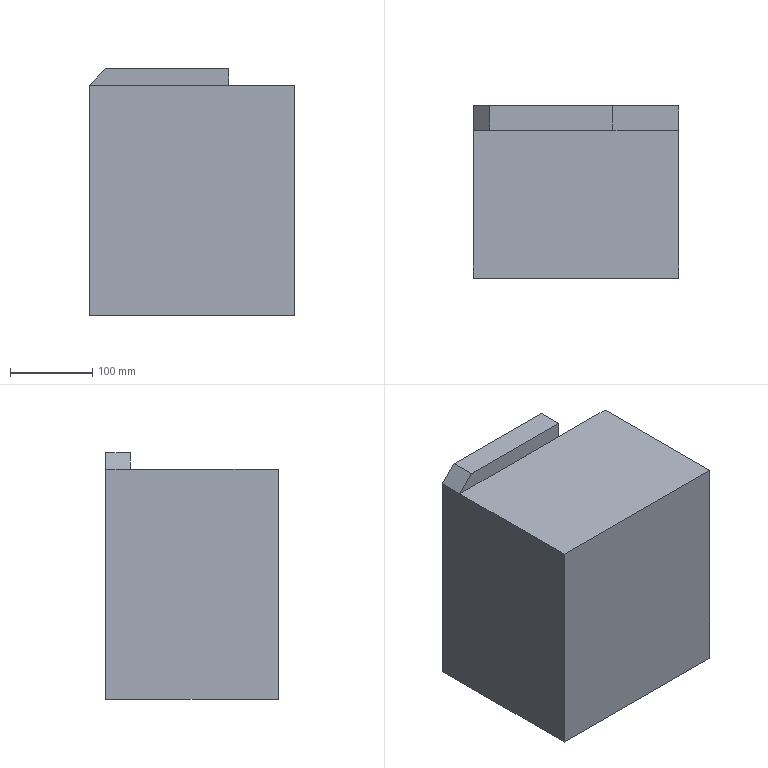Component | SolidWorks | -3[1]-1 | 1 solid | 15 faces | box 250 x 210 x 300 mm | volume 14226823 mm3 | plane 13 | cylinder 2 | commonest cylinder face diameters 27 x2
STEP:
#1=COLOUR_RGB('',0.7922,0.8196,0.9333);
#2=FILL_AREA_STYLE_COLOUR('',#1);
#3=FILL_AREA_STYLE('',(#2));
#4=SURFACE_STYLE_FILL_AREA(#3);
#5=SURFACE_SIDE_STYLE('',(#4));
#6=SURFACE_STYLE_USAGE(.BOTH.,#5);
#7=PRESENTATION_STYLE_ASSIGNMENT((#6));
#8=CARTESIAN_POINT('',(-19.685,-89.764,-4.39));
#9=VERTEX_POINT('',#8);
#10=CARTESIAN_POINT('',(-19.685,-89.764,-5.453));
#11=VERTEX_POINT('',#10);
#12=CARTESIAN_POINT('',(-19.685,-89.764,-4.921));
#13=DIRECTION('',(0.,-1.,0.));
#14=DIRECTION('',(0.,0.,-1.));
#15=AXIS2_PLACEMENT_3D('',#12,#13,#14);
#16=CIRCLE('',#15,0.5315);
#17=EDGE_CURVE('',#9,#11,#16,.T.);
#18=ORIENTED_EDGE('',*,*,#17,.T.);
#19=CARTESIAN_POINT('',(-19.685,-88.583,-5.453));
#20=VERTEX_POINT('',#19);
#21=CARTESIAN_POINT('',(-19.685,-89.764,-5.453));
#22=DIRECTION('',(0.,1.,0.));
#23=VECTOR('',#22,39.37);
#24=LINE('',#21,#23);
#25=EDGE_CURVE('',#11,#20,#24,.T.);
#26=ORIENTED_EDGE('',*,*,#25,.T.);
#27=CARTESIAN_POINT('',(-19.685,-88.583,-4.39));
#28=VERTEX_POINT('',#27);
#29=CARTESIAN_POINT('',(-19.685,-88.583,-4.921));
#30=DIRECTION('',(0.,-1.,0.));
#31=DIRECTION('',(0.,0.,-1.));
#32=AXIS2_PLACEMENT_3D('',#29,#30,#31);
#33=CIRCLE('',#32,0.5315);
#34=EDGE_CURVE('',#28,#20,#33,.T.);
#35=ORIENTED_EDGE('',*,*,#34,.F.);
#36=CARTESIAN_POINT('',(-19.685,-89.764,-4.39));
#37=DIRECTION('',(0.,1.,0.));
#38=VECTOR('',#37,39.37);
#39=LINE('',#36,#38);
#40=EDGE_CURVE('',#9,#28,#39,.T.);
#41=ORIENTED_EDGE('',*,*,#40,.F.);
#42=EDGE_LOOP('',(#18,#26,#35,#41));
#43=FACE_OUTER_BOUND('',#42,.T.);
#44=CARTESIAN_POINT('',(-19.685,-89.764,-4.921));
#45=DIRECTION('',(0.,1.,0.));
#46=DIRECTION('',(0.,0.,-1.));
#47=AXIS2_PLACEMENT_3D('',#44,#45,#46);
#48=CYLINDRICAL_SURFACE('',#47,0.5315);
#49=ADVANCED_FACE('',(#43),#48,.F.);
#50=CARTESIAN_POINT('',(-14.961,-89.764,2.165));
#51=VERTEX_POINT('',#50);
#52=CARTESIAN_POINT('',(-21.654,-89.764,2.165));
#53=VERTEX_POINT('',#52);
#54=CARTESIAN_POINT('',(-21.654,-89.764,2.165));
#55=DIRECTION('',(-1.,0.,0.));
#56=VECTOR('',#55,39.37);
#57=LINE('',#54,#56);
#58=EDGE_CURVE('',#51,#53,#57,.T.);
#59=ORIENTED_EDGE('',*,*,#58,.F.);
#60=CARTESIAN_POINT('',(-14.961,-89.764,2.953));
#61=VERTEX_POINT('',#60);
#62=CARTESIAN_POINT('',(-14.961,-89.764,2.953));
#63=DIRECTION('',(-0.,0.,1.));
#64=VECTOR('',#63,39.37);
#65=LINE('',#62,#64);
#66=EDGE_CURVE('',#51,#61,#65,.T.);
#67=ORIENTED_EDGE('',*,*,#66,.T.);
#68=CARTESIAN_POINT('',(-20.866,-89.764,2.953));
#69=VERTEX_POINT('',#68);
#70=CARTESIAN_POINT('',(-20.866,-89.764,2.953));
#71=DIRECTION('',(-1.,0.,0.));
#72=VECTOR('',#71,39.37);
#73=LINE('',#70,#72);
#74=EDGE_CURVE('',#61,#69,#73,.T.);
#75=ORIENTED_EDGE('',*,*,#74,.T.);
#76=CARTESIAN_POINT('',(-21.654,-89.764,2.165));
#77=DIRECTION('',(-0.7071,0.,-0.7071));
#78=VECTOR('',#77,39.37);
#79=LINE('',#76,#78);
#80=EDGE_CURVE('',#69,#53,#79,.T.);
#81=ORIENTED_EDGE('',*,*,#80,.T.);
#82=EDGE_LOOP('',(#59,#67,#75,#81));
#83=FACE_OUTER_BOUND('',#82,.T.);
#84=CARTESIAN_POINT('',(-21.654,-89.764,-8.858));
#85=DIRECTION('',(0.,1.,0.));
#86=DIRECTION('',(0.,0.,-1.));
#87=AXIS2_PLACEMENT_3D('',#84,#85,#86);
#88=PLANE('',#87);
#89=ADVANCED_FACE('',(#83),#88,.F.);
#90=CARTESIAN_POINT('',(-21.654,-88.583,-8.858));
#91=VERTEX_POINT('',#90);
#92=CARTESIAN_POINT('',(-11.811,-88.583,-8.858));
#93=VERTEX_POINT('',#92);
#94=CARTESIAN_POINT('',(-11.811,-88.583,-8.858));
#95=DIRECTION('',(1.,0.,0.));
#96=VECTOR('',#95,39.37);
#97=LINE('',#94,#96);
#98=EDGE_CURVE('',#91,#93,#97,.T.);
#99=ORIENTED_EDGE('',*,*,#98,.F.);
#100=CARTESIAN_POINT('',(-21.654,-88.583,2.165));
#101=VERTEX_POINT('',#100);
#102=CARTESIAN_POINT('',(-21.654,-88.583,-8.858));
#103=DIRECTION('',(0.,0.,-1.));
#104=VECTOR('',#103,39.37);
#105=LINE('',#102,#104);
#106=EDGE_CURVE('',#101,#91,#105,.T.);
#107=ORIENTED_EDGE('',*,*,#106,.F.);
#108=CARTESIAN_POINT('',(-20.866,-88.583,2.953));
#109=VERTEX_POINT('',#108);
#110=CARTESIAN_POINT('',(-21.654,-88.583,2.165));
#111=DIRECTION('',(-0.7071,0.,-0.7071));
#112=VECTOR('',#111,39.37);
#113=LINE('',#110,#112);
#114=EDGE_CURVE('',#109,#101,#113,.T.);
#115=ORIENTED_EDGE('',*,*,#114,.F.);
#116=CARTESIAN_POINT('',(-14.961,-88.583,2.953));
#117=VERTEX_POINT('',#116);
#118=CARTESIAN_POINT('',(-20.866,-88.583,2.953));
#119=DIRECTION('',(-1.,0.,0.));
#120=VECTOR('',#119,39.37);
#121=LINE('',#118,#120);
#122=EDGE_CURVE('',#117,#109,#121,.T.);
#123=ORIENTED_EDGE('',*,*,#122,.F.);
#124=CARTESIAN_POINT('',(-14.961,-88.583,-6.89));
#125=VERTEX_POINT('',#124);
#126=CARTESIAN_POINT('',(-14.961,-88.583,2.953));
#127=DIRECTION('',(-0.,0.,1.));
#128=VECTOR('',#127,39.37);
#129=LINE('',#126,#128);
#130=EDGE_CURVE('',#125,#117,#129,.T.);
#131=ORIENTED_EDGE('',*,*,#130,.F.);
#132=CARTESIAN_POINT('',(-11.811,-88.583,-6.89));
#133=VERTEX_POINT('',#132);
#134=CARTESIAN_POINT('',(-14.961,-88.583,-6.89));
#135=DIRECTION('',(-1.,0.,0.));
#136=VECTOR('',#135,39.37);
#137=LINE('',#134,#136);
#138=EDGE_CURVE('',#133,#125,#137,.T.);
#139=ORIENTED_EDGE('',*,*,#138,.F.);
#140=CARTESIAN_POINT('',(-11.811,-88.583,-6.89));
#141=DIRECTION('',(0.,0.,1.));
#142=VECTOR('',#141,39.37);
#143=LINE('',#140,#142);
#144=EDGE_CURVE('',#93,#133,#143,.T.);
#145=ORIENTED_EDGE('',*,*,#144,.F.);
#146=EDGE_LOOP('',(#99,#107,#115,#123,#131,#139,#145));
#147=FACE_OUTER_BOUND('',#146,.T.);
#148=ORIENTED_EDGE('',*,*,#34,.T.);
#149=CARTESIAN_POINT('',(-19.685,-88.583,-4.921));
#150=DIRECTION('',(0.,-1.,0.));
#151=DIRECTION('',(0.,0.,-1.));
#152=AXIS2_PLACEMENT_3D('',#149,#150,#151);
#153=CIRCLE('',#152,0.5315);
#154=EDGE_CURVE('',#20,#28,#153,.T.);
#155=ORIENTED_EDGE('',*,*,#154,.T.);
#156=EDGE_LOOP('',(#148,#155));
#157=FACE_BOUND('',#156,.T.);
#158=CARTESIAN_POINT('',(-21.654,-88.583,-8.858));
#159=DIRECTION('',(0.,1.,0.));
#160=DIRECTION('',(0.,0.,-1.));
#161=AXIS2_PLACEMENT_3D('',#158,#159,#160);
#162=PLANE('',#161);
#163=ADVANCED_FACE('',(#147,#157),#162,.T.);
#164=ORIENTED_EDGE('',*,*,#98,.T.);
#165=CARTESIAN_POINT('',(-11.811,-96.85,-8.858));
#166=VERTEX_POINT('',#165);
#167=CARTESIAN_POINT('',(-11.811,-89.764,-8.858));
#168=DIRECTION('',(0.,1.,0.));
#169=VECTOR('',#168,39.37);
#170=LINE('',#167,#169);
#171=EDGE_CURVE('',#166,#93,#170,.T.);
#172=ORIENTED_EDGE('',*,*,#171,.F.);
#173=CARTESIAN_POINT('',(-21.654,-96.85,-8.858));
#174=VERTEX_POINT('',#173);
#175=CARTESIAN_POINT('',(-21.654,-96.85,-8.858));
#176=DIRECTION('',(1.,0.,0.));
#177=VECTOR('',#176,39.37);
#178=LINE('',#175,#177);
#179=EDGE_CURVE('',#174,#166,#178,.T.);
#180=ORIENTED_EDGE('',*,*,#179,.F.);
#181=CARTESIAN_POINT('',(-21.654,-89.764,-8.858));
#182=DIRECTION('',(0.,1.,0.));
#183=VECTOR('',#182,39.37);
#184=LINE('',#181,#183);
#185=EDGE_CURVE('',#174,#91,#184,.T.);
#186=ORIENTED_EDGE('',*,*,#185,.T.);
#187=EDGE_LOOP('',(#164,#172,#180,#186));
#188=FACE_OUTER_BOUND('',#187,.T.);
#189=CARTESIAN_POINT('',(-11.811,-89.764,-8.858));
#190=DIRECTION('',(0.,0.,1.));
#191=DIRECTION('',(-1.,0.,0.));
#192=AXIS2_PLACEMENT_3D('',#189,#190,#191);
#193=PLANE('',#192);
#194=ADVANCED_FACE('',(#188),#193,.F.);
#195=ORIENTED_EDGE('',*,*,#144,.T.);
#196=CARTESIAN_POINT('',(-11.811,-89.764,-6.89));
#197=VERTEX_POINT('',#196);
#198=CARTESIAN_POINT('',(-11.811,-89.764,-6.89));
#199=DIRECTION('',(0.,1.,0.));
#200=VECTOR('',#199,39.37);
#201=LINE('',#198,#200);
#202=EDGE_CURVE('',#197,#133,#201,.T.);
#203=ORIENTED_EDGE('',*,*,#202,.F.);
#204=CARTESIAN_POINT('',(-11.811,-89.764,2.165));
#205=VERTEX_POINT('',#204);
#206=CARTESIAN_POINT('',(-11.811,-89.764,2.165));
#207=DIRECTION('',(0.,0.,1.));
#208=VECTOR('',#207,39.37);
#209=LINE('',#206,#208);
#210=EDGE_CURVE('',#197,#205,#209,.T.);
#211=ORIENTED_EDGE('',*,*,#210,.T.);
#212=CARTESIAN_POINT('',(-11.811,-96.85,2.165));
#213=VERTEX_POINT('',#212);
#214=CARTESIAN_POINT('',(-11.811,-96.85,2.165));
#215=DIRECTION('',(0.,1.,0.));
#216=VECTOR('',#215,39.37);
#217=LINE('',#214,#216);
#218=EDGE_CURVE('',#213,#205,#217,.T.);
#219=ORIENTED_EDGE('',*,*,#218,.F.);
#220=CARTESIAN_POINT('',(-11.811,-96.85,2.165));
#221=DIRECTION('',(0.,0.,1.));
#222=VECTOR('',#221,39.37);
#223=LINE('',#220,#222);
#224=EDGE_CURVE('',#166,#213,#223,.T.);
#225=ORIENTED_EDGE('',*,*,#224,.F.);
#226=ORIENTED_EDGE('',*,*,#171,.T.);
#227=EDGE_LOOP('',(#195,#203,#211,#219,#225,#226));
#228=FACE_OUTER_BOUND('',#227,.T.);
#229=CARTESIAN_POINT('',(-11.811,-89.764,-6.89));
#230=DIRECTION('',(-1.,0.,0.));
#231=DIRECTION('',(0.,0.,-1.));
#232=AXIS2_PLACEMENT_3D('',#229,#230,#231);
#233=PLANE('',#232);
#234=ADVANCED_FACE('',(#228),#233,.F.);
#235=ORIENTED_EDGE('',*,*,#138,.T.);
#236=CARTESIAN_POINT('',(-14.961,-89.764,-6.89));
#237=VERTEX_POINT('',#236);
#238=CARTESIAN_POINT('',(-14.961,-89.764,-6.89));
#239=DIRECTION('',(0.,1.,0.));
#240=VECTOR('',#239,39.37);
#241=LINE('',#238,#240);
#242=EDGE_CURVE('',#237,#125,#241,.T.);
#243=ORIENTED_EDGE('',*,*,#242,.F.);
#244=CARTESIAN_POINT('',(-14.961,-89.764,-6.89));
#245=DIRECTION('',(-1.,0.,0.));
#246=VECTOR('',#245,39.37);
#247=LINE('',#244,#246);
#248=EDGE_CURVE('',#197,#237,#247,.T.);
#249=ORIENTED_EDGE('',*,*,#248,.F.);
#250=ORIENTED_EDGE('',*,*,#202,.T.);
#251=EDGE_LOOP('',(#235,#243,#249,#250));
#252=FACE_OUTER_BOUND('',#251,.T.);
#253=CARTESIAN_POINT('',(-14.961,-89.764,-6.89));
#254=DIRECTION('',(0.,0.,-1.));
#255=DIRECTION('',(1.,0.,0.));
#256=AXIS2_PLACEMENT_3D('',#253,#254,#255);
#257=PLANE('',#256);
#258=ADVANCED_FACE('',(#252),#257,.F.);
#259=ORIENTED_EDGE('',*,*,#130,.T.);
#260=CARTESIAN_POINT('',(-14.961,-89.764,2.953));
#261=DIRECTION('',(0.,1.,0.));
#262=VECTOR('',#261,39.37);
#263=LINE('',#260,#262);
#264=EDGE_CURVE('',#61,#117,#263,.T.);
#265=ORIENTED_EDGE('',*,*,#264,.F.);
#266=ORIENTED_EDGE('',*,*,#66,.F.);
#267=CARTESIAN_POINT('',(-14.961,-89.764,2.953));
#268=DIRECTION('',(-0.,0.,1.));
#269=VECTOR('',#268,39.37);
#270=LINE('',#267,#269);
#271=EDGE_CURVE('',#237,#51,#270,.T.);
#272=ORIENTED_EDGE('',*,*,#271,.F.);
#273=ORIENTED_EDGE('',*,*,#242,.T.);
#274=EDGE_LOOP('',(#259,#265,#266,#272,#273));
#275=FACE_OUTER_BOUND('',#274,.T.);
#276=CARTESIAN_POINT('',(-14.961,-89.764,2.953));
#277=DIRECTION('',(-1.,0.,-0.));
#278=DIRECTION('',(0.,0.,-1.));
#279=AXIS2_PLACEMENT_3D('',#276,#277,#278);
#280=PLANE('',#279);
#281=ADVANCED_FACE('',(#275),#280,.F.);
#282=ORIENTED_EDGE('',*,*,#122,.T.);
#283=CARTESIAN_POINT('',(-20.866,-89.764,2.953));
#284=DIRECTION('',(0.,1.,0.));
#285=VECTOR('',#284,39.37);
#286=LINE('',#283,#285);
#287=EDGE_CURVE('',#69,#109,#286,.T.);
#288=ORIENTED_EDGE('',*,*,#287,.F.);
#289=ORIENTED_EDGE('',*,*,#74,.F.);
#290=ORIENTED_EDGE('',*,*,#264,.T.);
#291=EDGE_LOOP('',(#282,#288,#289,#290));
#292=FACE_OUTER_BOUND('',#291,.T.);
#293=CARTESIAN_POINT('',(-20.866,-89.764,2.953));
#294=DIRECTION('',(0.,0.,-1.));
#295=DIRECTION('',(1.,0.,0.));
#296=AXIS2_PLACEMENT_3D('',#293,#294,#295);
#297=PLANE('',#296);
#298=ADVANCED_FACE('',(#292),#297,.F.);
#299=ORIENTED_EDGE('',*,*,#114,.T.);
#300=CARTESIAN_POINT('',(-21.654,-89.764,2.165));
#301=DIRECTION('',(0.,1.,0.));
#302=VECTOR('',#301,39.37);
#303=LINE('',#300,#302);
#304=EDGE_CURVE('',#53,#101,#303,.T.);
#305=ORIENTED_EDGE('',*,*,#304,.F.);
#306=ORIENTED_EDGE('',*,*,#80,.F.);
#307=ORIENTED_EDGE('',*,*,#287,.T.);
#308=EDGE_LOOP('',(#299,#305,#306,#307));
#309=FACE_OUTER_BOUND('',#308,.T.);
#310=CARTESIAN_POINT('',(-21.654,-89.764,2.165));
#311=DIRECTION('',(0.7071,0.,-0.7071));
#312=DIRECTION('',(0.7071,0.,0.7071));
#313=AXIS2_PLACEMENT_3D('',#310,#311,#312);
#314=PLANE('',#313);
#315=ADVANCED_FACE('',(#309),#314,.F.);
#316=ORIENTED_EDGE('',*,*,#106,.T.);
#317=ORIENTED_EDGE('',*,*,#185,.F.);
#318=CARTESIAN_POINT('',(-21.654,-96.85,2.165));
#319=VERTEX_POINT('',#318);
#320=CARTESIAN_POINT('',(-21.654,-96.85,2.165));
#321=DIRECTION('',(0.,0.,-1.));
#322=VECTOR('',#321,39.37);
#323=LINE('',#320,#322);
#324=EDGE_CURVE('',#319,#174,#323,.T.);
#325=ORIENTED_EDGE('',*,*,#324,.F.);
#326=CARTESIAN_POINT('',(-21.654,-96.85,2.165));
#327=DIRECTION('',(0.,1.,0.));
#328=VECTOR('',#327,39.37);
#329=LINE('',#326,#328);
#330=EDGE_CURVE('',#319,#53,#329,.T.);
#331=ORIENTED_EDGE('',*,*,#330,.T.);
#332=ORIENTED_EDGE('',*,*,#304,.T.);
#333=EDGE_LOOP('',(#316,#317,#325,#331,#332));
#334=FACE_OUTER_BOUND('',#333,.T.);
#335=CARTESIAN_POINT('',(-21.654,-89.764,-8.858));
#336=DIRECTION('',(1.,0.,0.));
#337=DIRECTION('',(0.,0.,1.));
#338=AXIS2_PLACEMENT_3D('',#335,#336,#337);
#339=PLANE('',#338);
#340=ADVANCED_FACE('',(#334),#339,.F.);
#341=ORIENTED_EDGE('',*,*,#25,.F.);
#342=CARTESIAN_POINT('',(-19.685,-89.764,-4.921));
#343=DIRECTION('',(0.,-1.,0.));
#344=DIRECTION('',(0.,0.,-1.));
#345=AXIS2_PLACEMENT_3D('',#342,#343,#344);
#346=CIRCLE('',#345,0.5315);
#347=EDGE_CURVE('',#11,#9,#346,.T.);
#348=ORIENTED_EDGE('',*,*,#347,.T.);
#349=ORIENTED_EDGE('',*,*,#40,.T.);
#350=ORIENTED_EDGE('',*,*,#154,.F.);
#351=EDGE_LOOP('',(#341,#348,#349,#350));
#352=FACE_OUTER_BOUND('',#351,.T.);
#353=CARTESIAN_POINT('',(-19.685,-89.764,-4.921));
#354=DIRECTION('',(0.,1.,0.));
#355=DIRECTION('',(0.,0.,-1.));
#356=AXIS2_PLACEMENT_3D('',#353,#354,#355);
#357=CYLINDRICAL_SURFACE('',#356,0.5315);
#358=ADVANCED_FACE('',(#352),#357,.F.);
#359=ORIENTED_EDGE('',*,*,#324,.T.);
#360=ORIENTED_EDGE('',*,*,#179,.T.);
#361=ORIENTED_EDGE('',*,*,#224,.T.);
#362=CARTESIAN_POINT('',(-21.654,-96.85,2.165));
#363=DIRECTION('',(-1.,0.,0.));
#364=VECTOR('',#363,39.37);
#365=LINE('',#362,#364);
#366=EDGE_CURVE('',#213,#319,#365,.T.);
#367=ORIENTED_EDGE('',*,*,#366,.T.);
#368=EDGE_LOOP('',(#359,#360,#361,#367));
#369=FACE_OUTER_BOUND('',#368,.T.);
#370=CARTESIAN_POINT('',(0.,-96.85,0.));
#371=DIRECTION('',(0.,-1.,0.));
#372=DIRECTION('',(0.,0.,1.));
#373=AXIS2_PLACEMENT_3D('',#370,#371,#372);
#374=PLANE('',#373);
#375=ADVANCED_FACE('',(#369),#374,.T.);
#376=CARTESIAN_POINT('',(-21.654,-89.764,2.165));
#377=DIRECTION('',(-1.,0.,0.));
#378=VECTOR('',#377,39.37);
#379=LINE('',#376,#378);
#380=EDGE_CURVE('',#205,#51,#379,.T.);
#381=ORIENTED_EDGE('',*,*,#380,.T.);
#382=ORIENTED_EDGE('',*,*,#58,.T.);
#383=ORIENTED_EDGE('',*,*,#330,.F.);
#384=ORIENTED_EDGE('',*,*,#366,.F.);
#385=ORIENTED_EDGE('',*,*,#218,.T.);
#386=EDGE_LOOP('',(#381,#382,#383,#384,#385));
#387=FACE_OUTER_BOUND('',#386,.T.);
#388=CARTESIAN_POINT('',(-21.654,-96.85,2.165));
#389=DIRECTION('',(0.,0.,-1.));
#390=DIRECTION('',(1.,0.,0.));
#391=AXIS2_PLACEMENT_3D('',#388,#389,#390);
#392=PLANE('',#391);
#393=ADVANCED_FACE('',(#387),#392,.F.);
#394=ORIENTED_EDGE('',*,*,#210,.F.);
#395=ORIENTED_EDGE('',*,*,#248,.T.);
#396=ORIENTED_EDGE('',*,*,#271,.T.);
#397=ORIENTED_EDGE('',*,*,#380,.F.);
#398=EDGE_LOOP('',(#394,#395,#396,#397));
#399=FACE_OUTER_BOUND('',#398,.T.);
#400=CARTESIAN_POINT('',(0.,-89.764,0.));
#401=DIRECTION('',(0.,-1.,0.));
#402=DIRECTION('',(0.,0.,1.));
#403=AXIS2_PLACEMENT_3D('',#400,#401,#402);
#404=PLANE('',#403);
#405=ADVANCED_FACE('',(#399),#404,.F.);
#406=ORIENTED_EDGE('',*,*,#17,.F.);
#407=ORIENTED_EDGE('',*,*,#347,.F.);
#408=EDGE_LOOP('',(#406,#407));
#409=FACE_OUTER_BOUND('',#408,.T.);
#410=CARTESIAN_POINT('',(0.,-89.764,0.));
#411=DIRECTION('',(0.,-1.,0.));
#412=DIRECTION('',(0.,0.,1.));
#413=AXIS2_PLACEMENT_3D('',#410,#411,#412);
#414=PLANE('',#413);
#415=ADVANCED_FACE('',(#409),#414,.F.);
#416=CLOSED_SHELL('',(#49,#89,#163,#194,#234,#258,#281,#298,#315,#340,#358,#375,#393,#405,#415));
#417=MANIFOLD_SOLID_BREP('',#416);
#418=STYLED_ITEM('',(#7),#417);
#419=PRESENTATION_LAYER_ASSIGNMENT('','',(#418));
#420=(LENGTH_UNIT()NAMED_UNIT(*)SI_UNIT($,.METRE.));
#421=LENGTH_MEASURE_WITH_UNIT(LENGTH_MEASURE(0.0254),#420);
#422=DIMENSIONAL_EXPONENTS(1.,0.,0.,0.,0.,0.,0.);
#423=(CONVERSION_BASED_UNIT('',#421)LENGTH_UNIT()NAMED_UNIT(#422));
#424=UNCERTAINTY_MEASURE_WITH_UNIT(LENGTH_MEASURE(0.00001),#423,'','');
#425=(NAMED_UNIT(*)PLANE_ANGLE_UNIT()SI_UNIT($,.RADIAN.));
#426=(NAMED_UNIT(*)SI_UNIT($,.STERADIAN.)SOLID_ANGLE_UNIT());
#427=(GEOMETRIC_REPRESENTATION_CONTEXT(3)GLOBAL_UNCERTAINTY_ASSIGNED_CONTEXT((#424))GLOBAL_UNIT_ASSIGNED_CONTEXT((#423,#425,#426))REPRESENTATION_CONTEXT('',''));
#428=MECHANICAL_DESIGN_GEOMETRIC_PRESENTATION_REPRESENTATION('',(#418),#427);
#429=CARTESIAN_POINT('',(0.,0.,0.));
#430=DIRECTION('',(0.,0.,1.));
#431=DIRECTION('',(1.,0.,0.));
#432=AXIS2_PLACEMENT_3D('',#429,#430,#431);
#433=(LENGTH_UNIT()NAMED_UNIT(*)SI_UNIT($,.METRE.));
#434=LENGTH_MEASURE_WITH_UNIT(LENGTH_MEASURE(0.0254),#433);
#435=DIMENSIONAL_EXPONENTS(1.,0.,0.,0.,0.,0.,0.);
#436=(CONVERSION_BASED_UNIT('',#434)LENGTH_UNIT()NAMED_UNIT(#435));
#437=UNCERTAINTY_MEASURE_WITH_UNIT(LENGTH_MEASURE(0.00001),#436,'','');
#438=(NAMED_UNIT(*)PLANE_ANGLE_UNIT()SI_UNIT($,.RADIAN.));
#439=(NAMED_UNIT(*)SI_UNIT($,.STERADIAN.)SOLID_ANGLE_UNIT());
#440=(GEOMETRIC_REPRESENTATION_CONTEXT(3)GLOBAL_UNCERTAINTY_ASSIGNED_CONTEXT((#437))GLOBAL_UNIT_ASSIGNED_CONTEXT((#436,#438,#439))REPRESENTATION_CONTEXT('',''));
#441=ADVANCED_BREP_SHAPE_REPRESENTATION('',(#417,#432),#440);